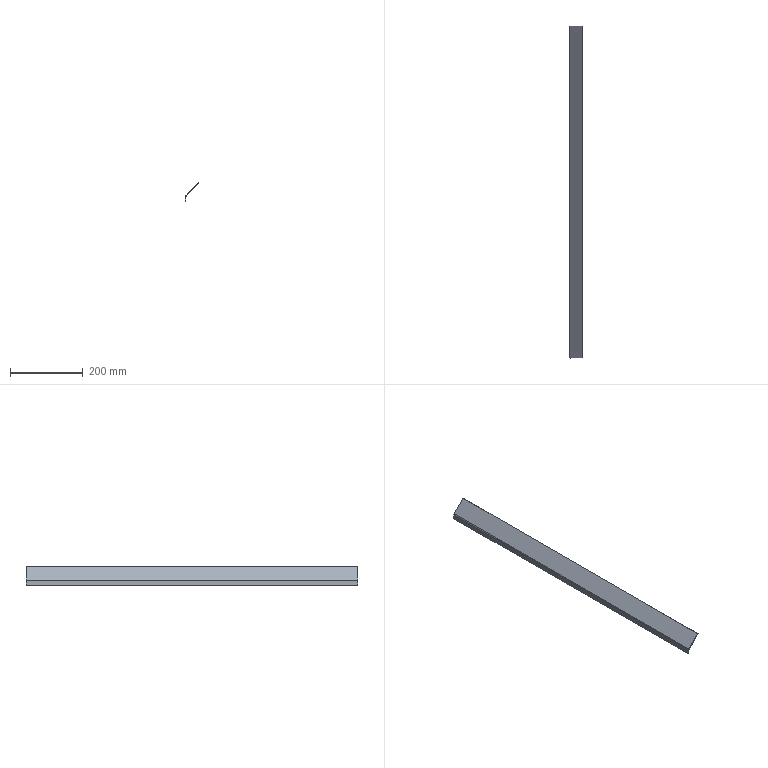Component | SolidWorks | ExhaustVentAssembly-1_Louver-1 | 1 solid | 16 faces | box 37.41 x 914 x 51 mm | volume 118659 mm3 | plane 14 | cylinder 2 | commonest cylinder face diameters 8 x1 4 x1 | material Plain Carbon Steel
STEP:
#1=CARTESIAN_POINT('',(-16.406,6.211,35.255));
#2=VERTEX_POINT('',#1);
#3=CARTESIAN_POINT('',(-16.406,42.1,35.255));
#4=VERTEX_POINT('',#3);
#5=CARTESIAN_POINT('',(-16.406,6.163,35.255));
#6=DIRECTION('',(0.,1.,-0.));
#7=VECTOR('',#6,39.37);
#8=LINE('',#5,#7);
#9=EDGE_CURVE('',#2,#4,#8,.T.);
#10=ORIENTED_EDGE('',*,*,#9,.F.);
#11=CARTESIAN_POINT('',(-16.485,6.211,35.255));
#12=VERTEX_POINT('',#11);
#13=CARTESIAN_POINT('',(-16.406,6.211,35.255));
#14=DIRECTION('',(-1.,0.,-0.));
#15=VECTOR('',#14,39.37);
#16=LINE('',#13,#15);
#17=EDGE_CURVE('',#2,#12,#16,.T.);
#18=ORIENTED_EDGE('',*,*,#17,.T.);
#19=CARTESIAN_POINT('',(-16.485,42.1,35.255));
#20=VERTEX_POINT('',#19);
#21=CARTESIAN_POINT('',(-16.485,6.163,35.255));
#22=DIRECTION('',(0.,1.,-0.));
#23=VECTOR('',#22,39.37);
#24=LINE('',#21,#23);
#25=EDGE_CURVE('',#12,#20,#24,.T.);
#26=ORIENTED_EDGE('',*,*,#25,.T.);
#27=CARTESIAN_POINT('',(-16.406,42.1,35.255));
#28=DIRECTION('',(1.,-0.,0.));
#29=VECTOR('',#28,39.37);
#30=LINE('',#27,#29);
#31=EDGE_CURVE('',#20,#4,#30,.T.);
#32=ORIENTED_EDGE('',*,*,#31,.T.);
#33=EDGE_LOOP('',(#10,#18,#26,#32));
#34=FACE_OUTER_BOUND('',#33,.T.);
#35=CARTESIAN_POINT('',(-16.406,6.163,35.255));
#36=DIRECTION('',(0.,-0.,-1.));
#37=DIRECTION('',(1.,-0.,0.));
#38=AXIS2_PLACEMENT_3D('',#35,#36,#37);
#39=PLANE('',#38);
#40=ADVANCED_FACE('',(#34),#39,.T.);
#41=CARTESIAN_POINT('',(-16.398,6.163,35.815));
#42=VERTEX_POINT('',#41);
#43=CARTESIAN_POINT('',(-16.398,6.163,35.851));
#44=VERTEX_POINT('',#43);
#45=CARTESIAN_POINT('',(-16.398,6.163,35.892));
#46=DIRECTION('',(-0.,0.,1.));
#47=VECTOR('',#46,39.37);
#48=LINE('',#45,#47);
#49=EDGE_CURVE('',#42,#44,#48,.T.);
#50=ORIENTED_EDGE('',*,*,#49,.F.);
#51=CARTESIAN_POINT('',(-16.383,6.163,35.836));
#52=VERTEX_POINT('',#51);
#53=CARTESIAN_POINT('',(-16.327,6.163,35.78));
#54=DIRECTION('',(0.,1.,-0.));
#55=DIRECTION('',(1.,0.,0.));
#56=AXIS2_PLACEMENT_3D('',#53,#54,#55);
#57=CIRCLE('',#56,0.07874);
#58=EDGE_CURVE('',#42,#52,#57,.T.);
#59=ORIENTED_EDGE('',*,*,#58,.T.);
#60=CARTESIAN_POINT('',(-16.439,6.163,35.892));
#61=DIRECTION('',(0.7071,-0.,-0.7071));
#62=VECTOR('',#61,39.37);
#63=LINE('',#60,#62);
#64=EDGE_CURVE('',#44,#52,#63,.T.);
#65=ORIENTED_EDGE('',*,*,#64,.F.);
#66=EDGE_LOOP('',(#50,#59,#65));
#67=FACE_OUTER_BOUND('',#66,.T.);
#68=CARTESIAN_POINT('',(-16.439,6.163,35.892));
#69=DIRECTION('',(-0.,-1.,0.));
#70=DIRECTION('',(1.,-0.,0.));
#71=AXIS2_PLACEMENT_3D('',#68,#69,#70);
#72=PLANE('',#71);
#73=ADVANCED_FACE('',(#67),#72,.T.);
#74=CARTESIAN_POINT('',(-16.398,6.163,35.932));
#75=VERTEX_POINT('',#74);
#76=CARTESIAN_POINT('',(-16.398,6.163,35.78));
#77=DIRECTION('',(-0.,0.,1.));
#78=VECTOR('',#77,39.37);
#79=LINE('',#76,#78);
#80=EDGE_CURVE('',#44,#75,#79,.T.);
#81=ORIENTED_EDGE('',*,*,#80,.F.);
#82=ORIENTED_EDGE('',*,*,#64,.T.);
#83=CARTESIAN_POINT('',(-15.012,6.163,37.207));
#84=VERTEX_POINT('',#83);
#85=CARTESIAN_POINT('',(-16.429,6.163,35.79));
#86=DIRECTION('',(0.7071,0.,0.7071));
#87=VECTOR('',#86,39.37);
#88=LINE('',#85,#87);
#89=EDGE_CURVE('',#52,#84,#88,.T.);
#90=ORIENTED_EDGE('',*,*,#89,.T.);
#91=CARTESIAN_POINT('',(-15.067,6.163,37.263));
#92=VERTEX_POINT('',#91);
#93=CARTESIAN_POINT('',(-15.067,6.163,37.263));
#94=DIRECTION('',(0.7071,-0.,-0.7071));
#95=VECTOR('',#94,39.37);
#96=LINE('',#93,#95);
#97=EDGE_CURVE('',#92,#84,#96,.T.);
#98=ORIENTED_EDGE('',*,*,#97,.F.);
#99=CARTESIAN_POINT('',(-16.485,6.163,35.846));
#100=DIRECTION('',(0.7071,0.,0.7071));
#101=VECTOR('',#100,39.37);
#102=LINE('',#99,#101);
#103=EDGE_CURVE('',#75,#92,#102,.T.);
#104=ORIENTED_EDGE('',*,*,#103,.F.);
#105=EDGE_LOOP('',(#81,#82,#90,#98,#104));
#106=FACE_OUTER_BOUND('',#105,.T.);
#107=CARTESIAN_POINT('',(-16.406,6.163,35.78));
#108=DIRECTION('',(-0.,-1.,0.));
#109=DIRECTION('',(1.,-0.,0.));
#110=AXIS2_PLACEMENT_3D('',#107,#108,#109);
#111=PLANE('',#110);
#112=ADVANCED_FACE('',(#106),#111,.T.);
#113=CARTESIAN_POINT('',(-16.398,42.148,35.851));
#114=VERTEX_POINT('',#113);
#115=CARTESIAN_POINT('',(-16.398,42.148,35.815));
#116=VERTEX_POINT('',#115);
#117=CARTESIAN_POINT('',(-16.398,42.148,35.78));
#118=DIRECTION('',(0.,-0.,-1.));
#119=VECTOR('',#118,39.37);
#120=LINE('',#117,#119);
#121=EDGE_CURVE('',#114,#116,#120,.T.);
#122=ORIENTED_EDGE('',*,*,#121,.F.);
#123=CARTESIAN_POINT('',(-16.383,42.148,35.836));
#124=VERTEX_POINT('',#123);
#125=CARTESIAN_POINT('',(-16.383,42.148,35.836));
#126=DIRECTION('',(-0.7071,0.,0.7071));
#127=VECTOR('',#126,39.37);
#128=LINE('',#125,#127);
#129=EDGE_CURVE('',#124,#114,#128,.T.);
#130=ORIENTED_EDGE('',*,*,#129,.F.);
#131=CARTESIAN_POINT('',(-16.327,42.148,35.78));
#132=DIRECTION('',(0.,1.,-0.));
#133=DIRECTION('',(1.,0.,0.));
#134=AXIS2_PLACEMENT_3D('',#131,#132,#133);
#135=CIRCLE('',#134,0.07874);
#136=EDGE_CURVE('',#116,#124,#135,.T.);
#137=ORIENTED_EDGE('',*,*,#136,.F.);
#138=EDGE_LOOP('',(#122,#130,#137));
#139=FACE_OUTER_BOUND('',#138,.T.);
#140=CARTESIAN_POINT('',(-16.485,42.148,35.78));
#141=DIRECTION('',(0.,1.,-0.));
#142=DIRECTION('',(-1.,0.,-0.));
#143=AXIS2_PLACEMENT_3D('',#140,#141,#142);
#144=PLANE('',#143);
#145=ADVANCED_FACE('',(#139),#144,.T.);
#146=CARTESIAN_POINT('',(-15.012,42.148,37.207));
#147=VERTEX_POINT('',#146);
#148=CARTESIAN_POINT('',(-16.429,42.148,35.79));
#149=DIRECTION('',(0.7071,0.,0.7071));
#150=VECTOR('',#149,39.37);
#151=LINE('',#148,#150);
#152=EDGE_CURVE('',#124,#147,#151,.T.);
#153=ORIENTED_EDGE('',*,*,#152,.T.);
#154=CARTESIAN_POINT('',(-15.012,6.163,37.207));
#155=DIRECTION('',(0.,1.,-0.));
#156=VECTOR('',#155,39.37);
#157=LINE('',#154,#156);
#158=EDGE_CURVE('',#84,#147,#157,.T.);
#159=ORIENTED_EDGE('',*,*,#158,.F.);
#160=ORIENTED_EDGE('',*,*,#89,.F.);
#161=CARTESIAN_POINT('',(-16.383,6.163,35.836));
#162=DIRECTION('',(0.,1.,-0.));
#163=VECTOR('',#162,39.37);
#164=LINE('',#161,#163);
#165=EDGE_CURVE('',#52,#124,#164,.T.);
#166=ORIENTED_EDGE('',*,*,#165,.T.);
#167=EDGE_LOOP('',(#153,#159,#160,#166));
#168=FACE_OUTER_BOUND('',#167,.T.);
#169=CARTESIAN_POINT('',(-16.429,6.163,35.79));
#170=DIRECTION('',(-0.7071,0.,0.7071));
#171=DIRECTION('',(-0.7071,-0.,-0.7071));
#172=AXIS2_PLACEMENT_3D('',#169,#170,#171);
#173=PLANE('',#172);
#174=ADVANCED_FACE('',(#168),#173,.F.);
#175=CARTESIAN_POINT('',(-15.067,42.148,37.263));
#176=VERTEX_POINT('',#175);
#177=CARTESIAN_POINT('',(-15.067,42.148,37.263));
#178=DIRECTION('',(0.7071,-0.,-0.7071));
#179=VECTOR('',#178,39.37);
#180=LINE('',#177,#179);
#181=EDGE_CURVE('',#176,#147,#180,.T.);
#182=ORIENTED_EDGE('',*,*,#181,.F.);
#183=CARTESIAN_POINT('',(-15.067,6.163,37.263));
#184=DIRECTION('',(0.,1.,-0.));
#185=VECTOR('',#184,39.37);
#186=LINE('',#183,#185);
#187=EDGE_CURVE('',#92,#176,#186,.T.);
#188=ORIENTED_EDGE('',*,*,#187,.F.);
#189=ORIENTED_EDGE('',*,*,#97,.T.);
#190=ORIENTED_EDGE('',*,*,#158,.T.);
#191=EDGE_LOOP('',(#182,#188,#189,#190));
#192=FACE_OUTER_BOUND('',#191,.T.);
#193=CARTESIAN_POINT('',(-15.067,6.163,37.263));
#194=DIRECTION('',(0.7071,0.,0.7071));
#195=DIRECTION('',(-0.7071,0.,0.7071));
#196=AXIS2_PLACEMENT_3D('',#193,#194,#195);
#197=PLANE('',#196);
#198=ADVANCED_FACE('',(#192),#197,.T.);
#199=CARTESIAN_POINT('',(-16.398,6.211,35.932));
#200=VERTEX_POINT('',#199);
#201=CARTESIAN_POINT('',(-16.439,6.211,35.892));
#202=VERTEX_POINT('',#201);
#203=CARTESIAN_POINT('',(-16.485,6.211,35.846));
#204=DIRECTION('',(-0.7071,-0.,-0.7071));
#205=VECTOR('',#204,39.37);
#206=LINE('',#203,#205);
#207=EDGE_CURVE('',#200,#202,#206,.T.);
#208=ORIENTED_EDGE('',*,*,#207,.F.);
#209=CARTESIAN_POINT('',(-16.398,6.163,35.932));
#210=DIRECTION('',(0.,1.,-0.));
#211=VECTOR('',#210,39.37);
#212=LINE('',#209,#211);
#213=EDGE_CURVE('',#75,#200,#212,.T.);
#214=ORIENTED_EDGE('',*,*,#213,.F.);
#215=ORIENTED_EDGE('',*,*,#103,.T.);
#216=ORIENTED_EDGE('',*,*,#187,.T.);
#217=CARTESIAN_POINT('',(-16.398,42.148,35.932));
#218=VERTEX_POINT('',#217);
#219=CARTESIAN_POINT('',(-16.485,42.148,35.846));
#220=DIRECTION('',(0.7071,0.,0.7071));
#221=VECTOR('',#220,39.37);
#222=LINE('',#219,#221);
#223=EDGE_CURVE('',#218,#176,#222,.T.);
#224=ORIENTED_EDGE('',*,*,#223,.F.);
#225=CARTESIAN_POINT('',(-16.398,42.1,35.932));
#226=VERTEX_POINT('',#225);
#227=CARTESIAN_POINT('',(-16.398,6.163,35.932));
#228=DIRECTION('',(0.,1.,-0.));
#229=VECTOR('',#228,39.37);
#230=LINE('',#227,#229);
#231=EDGE_CURVE('',#226,#218,#230,.T.);
#232=ORIENTED_EDGE('',*,*,#231,.F.);
#233=CARTESIAN_POINT('',(-16.439,42.1,35.892));
#234=VERTEX_POINT('',#233);
#235=CARTESIAN_POINT('',(-16.485,42.1,35.846));
#236=DIRECTION('',(0.7071,0.,0.7071));
#237=VECTOR('',#236,39.37);
#238=LINE('',#235,#237);
#239=EDGE_CURVE('',#234,#226,#238,.T.);
#240=ORIENTED_EDGE('',*,*,#239,.F.);
#241=CARTESIAN_POINT('',(-16.439,6.163,35.892));
#242=DIRECTION('',(0.,1.,-0.));
#243=VECTOR('',#242,39.37);
#244=LINE('',#241,#243);
#245=EDGE_CURVE('',#202,#234,#244,.T.);
#246=ORIENTED_EDGE('',*,*,#245,.F.);
#247=EDGE_LOOP('',(#208,#214,#215,#216,#224,#232,#240,#246));
#248=FACE_OUTER_BOUND('',#247,.T.);
#249=CARTESIAN_POINT('',(-16.485,6.163,35.846));
#250=DIRECTION('',(-0.7071,0.,0.7071));
#251=DIRECTION('',(-0.7071,-0.,-0.7071));
#252=AXIS2_PLACEMENT_3D('',#249,#250,#251);
#253=PLANE('',#252);
#254=ADVANCED_FACE('',(#248),#253,.T.);
#255=CARTESIAN_POINT('',(-16.485,6.211,35.78));
#256=VERTEX_POINT('',#255);
#257=CARTESIAN_POINT('',(-16.327,6.211,35.78));
#258=DIRECTION('',(-0.,-1.,0.));
#259=DIRECTION('',(-1.,0.,0.));
#260=AXIS2_PLACEMENT_3D('',#257,#258,#259);
#261=CIRCLE('',#260,0.1575);
#262=EDGE_CURVE('',#202,#256,#261,.T.);
#263=ORIENTED_EDGE('',*,*,#262,.F.);
#264=ORIENTED_EDGE('',*,*,#245,.T.);
#265=CARTESIAN_POINT('',(-16.485,42.1,35.78));
#266=VERTEX_POINT('',#265);
#267=CARTESIAN_POINT('',(-16.327,42.1,35.78));
#268=DIRECTION('',(0.,1.,-0.));
#269=DIRECTION('',(1.,0.,0.));
#270=AXIS2_PLACEMENT_3D('',#267,#268,#269);
#271=CIRCLE('',#270,0.1575);
#272=EDGE_CURVE('',#266,#234,#271,.T.);
#273=ORIENTED_EDGE('',*,*,#272,.F.);
#274=CARTESIAN_POINT('',(-16.485,6.163,35.78));
#275=DIRECTION('',(0.,1.,-0.));
#276=VECTOR('',#275,39.37);
#277=LINE('',#274,#276);
#278=EDGE_CURVE('',#256,#266,#277,.T.);
#279=ORIENTED_EDGE('',*,*,#278,.F.);
#280=EDGE_LOOP('',(#263,#264,#273,#279));
#281=FACE_OUTER_BOUND('',#280,.T.);
#282=CARTESIAN_POINT('',(-16.327,6.163,35.78));
#283=DIRECTION('',(0.,1.,-0.));
#284=DIRECTION('',(-1.,0.,0.));
#285=AXIS2_PLACEMENT_3D('',#282,#283,#284);
#286=CYLINDRICAL_SURFACE('',#285,0.1575);
#287=ADVANCED_FACE('',(#281),#286,.T.);
#288=CARTESIAN_POINT('',(-16.485,6.211,35.255));
#289=DIRECTION('',(0.,-0.,-1.));
#290=VECTOR('',#289,39.37);
#291=LINE('',#288,#290);
#292=EDGE_CURVE('',#256,#12,#291,.T.);
#293=ORIENTED_EDGE('',*,*,#292,.F.);
#294=ORIENTED_EDGE('',*,*,#278,.T.);
#295=CARTESIAN_POINT('',(-16.485,42.1,35.255));
#296=DIRECTION('',(-0.,0.,1.));
#297=VECTOR('',#296,39.37);
#298=LINE('',#295,#297);
#299=EDGE_CURVE('',#20,#266,#298,.T.);
#300=ORIENTED_EDGE('',*,*,#299,.F.);
#301=ORIENTED_EDGE('',*,*,#25,.F.);
#302=EDGE_LOOP('',(#293,#294,#300,#301));
#303=FACE_OUTER_BOUND('',#302,.T.);
#304=CARTESIAN_POINT('',(-16.485,6.163,35.255));
#305=DIRECTION('',(-1.,0.,-0.));
#306=DIRECTION('',(-0.,-1.,0.));
#307=AXIS2_PLACEMENT_3D('',#304,#305,#306);
#308=PLANE('',#307);
#309=ADVANCED_FACE('',(#303),#308,.T.);
#310=CARTESIAN_POINT('',(-16.406,6.211,35.78));
#311=VERTEX_POINT('',#310);
#312=CARTESIAN_POINT('',(-16.406,42.1,35.78));
#313=VERTEX_POINT('',#312);
#314=CARTESIAN_POINT('',(-16.406,6.163,35.78));
#315=DIRECTION('',(0.,1.,-0.));
#316=VECTOR('',#315,39.37);
#317=LINE('',#314,#316);
#318=EDGE_CURVE('',#311,#313,#317,.T.);
#319=ORIENTED_EDGE('',*,*,#318,.F.);
#320=CARTESIAN_POINT('',(-16.406,6.211,35.255));
#321=DIRECTION('',(0.,-0.,-1.));
#322=VECTOR('',#321,39.37);
#323=LINE('',#320,#322);
#324=EDGE_CURVE('',#311,#2,#323,.T.);
#325=ORIENTED_EDGE('',*,*,#324,.T.);
#326=ORIENTED_EDGE('',*,*,#9,.T.);
#327=CARTESIAN_POINT('',(-16.406,42.1,35.255));
#328=DIRECTION('',(-0.,0.,1.));
#329=VECTOR('',#328,39.37);
#330=LINE('',#327,#329);
#331=EDGE_CURVE('',#4,#313,#330,.T.);
#332=ORIENTED_EDGE('',*,*,#331,.T.);
#333=EDGE_LOOP('',(#319,#325,#326,#332));
#334=FACE_OUTER_BOUND('',#333,.T.);
#335=CARTESIAN_POINT('',(-16.406,6.163,35.255));
#336=DIRECTION('',(-1.,0.,-0.));
#337=DIRECTION('',(-0.,-1.,0.));
#338=AXIS2_PLACEMENT_3D('',#335,#336,#337);
#339=PLANE('',#338);
#340=ADVANCED_FACE('',(#334),#339,.F.);
#341=CARTESIAN_POINT('',(-16.398,6.211,35.815));
#342=VERTEX_POINT('',#341);
#343=CARTESIAN_POINT('',(-16.398,6.163,35.815));
#344=DIRECTION('',(0.,1.,-0.));
#345=VECTOR('',#344,39.37);
#346=LINE('',#343,#345);
#347=EDGE_CURVE('',#42,#342,#346,.T.);
#348=ORIENTED_EDGE('',*,*,#347,.T.);
#349=CARTESIAN_POINT('',(-16.327,6.211,35.78));
#350=DIRECTION('',(-0.,-1.,0.));
#351=DIRECTION('',(-1.,0.,0.));
#352=AXIS2_PLACEMENT_3D('',#349,#350,#351);
#353=CIRCLE('',#352,0.07874);
#354=EDGE_CURVE('',#342,#311,#353,.T.);
#355=ORIENTED_EDGE('',*,*,#354,.T.);
#356=ORIENTED_EDGE('',*,*,#318,.T.);
#357=CARTESIAN_POINT('',(-16.398,42.1,35.815));
#358=VERTEX_POINT('',#357);
#359=CARTESIAN_POINT('',(-16.327,42.1,35.78));
#360=DIRECTION('',(0.,1.,-0.));
#361=DIRECTION('',(1.,0.,-0.));
#362=AXIS2_PLACEMENT_3D('',#359,#360,#361);
#363=CIRCLE('',#362,0.07874);
#364=EDGE_CURVE('',#313,#358,#363,.T.);
#365=ORIENTED_EDGE('',*,*,#364,.T.);
#366=CARTESIAN_POINT('',(-16.398,6.163,35.815));
#367=DIRECTION('',(0.,1.,-0.));
#368=VECTOR('',#367,39.37);
#369=LINE('',#366,#368);
#370=EDGE_CURVE('',#358,#116,#369,.T.);
#371=ORIENTED_EDGE('',*,*,#370,.T.);
#372=ORIENTED_EDGE('',*,*,#136,.T.);
#373=ORIENTED_EDGE('',*,*,#165,.F.);
#374=ORIENTED_EDGE('',*,*,#58,.F.);
#375=EDGE_LOOP('',(#348,#355,#356,#365,#371,#372,#373,#374));
#376=FACE_OUTER_BOUND('',#375,.T.);
#377=CARTESIAN_POINT('',(-16.327,6.163,35.78));
#378=DIRECTION('',(0.,1.,-0.));
#379=DIRECTION('',(-1.,0.,0.));
#380=AXIS2_PLACEMENT_3D('',#377,#378,#379);
#381=CYLINDRICAL_SURFACE('',#380,0.07874);
#382=ADVANCED_FACE('',(#376),#381,.F.);
#383=ORIENTED_EDGE('',*,*,#129,.T.);
#384=CARTESIAN_POINT('',(-16.398,42.148,35.78));
#385=DIRECTION('',(-0.,0.,1.));
#386=VECTOR('',#385,39.37);
#387=LINE('',#384,#386);
#388=EDGE_CURVE('',#114,#218,#387,.T.);
#389=ORIENTED_EDGE('',*,*,#388,.T.);
#390=ORIENTED_EDGE('',*,*,#223,.T.);
#391=ORIENTED_EDGE('',*,*,#181,.T.);
#392=ORIENTED_EDGE('',*,*,#152,.F.);
#393=EDGE_LOOP('',(#383,#389,#390,#391,#392));
#394=FACE_OUTER_BOUND('',#393,.T.);
#395=CARTESIAN_POINT('',(-16.327,42.148,35.78));
#396=DIRECTION('',(-0.,-1.,0.));
#397=DIRECTION('',(1.,-0.,0.));
#398=AXIS2_PLACEMENT_3D('',#395,#396,#397);
#399=PLANE('',#398);
#400=ADVANCED_FACE('',(#394),#399,.F.);
#401=ORIENTED_EDGE('',*,*,#239,.T.);
#402=CARTESIAN_POINT('',(-16.398,42.1,35.255));
#403=DIRECTION('',(-0.,0.,1.));
#404=VECTOR('',#403,39.37);
#405=LINE('',#402,#404);
#406=EDGE_CURVE('',#358,#226,#405,.T.);
#407=ORIENTED_EDGE('',*,*,#406,.F.);
#408=ORIENTED_EDGE('',*,*,#364,.F.);
#409=ORIENTED_EDGE('',*,*,#331,.F.);
#410=ORIENTED_EDGE('',*,*,#31,.F.);
#411=ORIENTED_EDGE('',*,*,#299,.T.);
#412=ORIENTED_EDGE('',*,*,#272,.T.);
#413=EDGE_LOOP('',(#401,#407,#408,#409,#410,#411,#412));
#414=FACE_OUTER_BOUND('',#413,.T.);
#415=CARTESIAN_POINT('',(-16.398,42.1,35.255));
#416=DIRECTION('',(-0.,-1.,0.));
#417=DIRECTION('',(1.,-0.,0.));
#418=AXIS2_PLACEMENT_3D('',#415,#416,#417);
#419=PLANE('',#418);
#420=ADVANCED_FACE('',(#414),#419,.F.);
#421=ORIENTED_EDGE('',*,*,#406,.T.);
#422=ORIENTED_EDGE('',*,*,#231,.T.);
#423=ORIENTED_EDGE('',*,*,#388,.F.);
#424=ORIENTED_EDGE('',*,*,#121,.T.);
#425=ORIENTED_EDGE('',*,*,#370,.F.);
#426=EDGE_LOOP('',(#421,#422,#423,#424,#425));
#427=FACE_OUTER_BOUND('',#426,.T.);
#428=CARTESIAN_POINT('',(-16.398,42.177,35.255));
#429=DIRECTION('',(1.,-0.,0.));
#430=DIRECTION('',(0.,1.,-0.));
#431=AXIS2_PLACEMENT_3D('',#428,#429,#430);
#432=PLANE('',#431);
#433=ADVANCED_FACE('',(#427),#432,.F.);
#434=ORIENTED_EDGE('',*,*,#207,.T.);
#435=ORIENTED_EDGE('',*,*,#262,.T.);
#436=ORIENTED_EDGE('',*,*,#292,.T.);
#437=ORIENTED_EDGE('',*,*,#17,.F.);
#438=ORIENTED_EDGE('',*,*,#324,.F.);
#439=ORIENTED_EDGE('',*,*,#354,.F.);
#440=CARTESIAN_POINT('',(-16.398,6.211,35.255));
#441=DIRECTION('',(-0.,0.,1.));
#442=VECTOR('',#441,39.37);
#443=LINE('',#440,#442);
#444=EDGE_CURVE('',#342,#200,#443,.T.);
#445=ORIENTED_EDGE('',*,*,#444,.T.);
#446=EDGE_LOOP('',(#434,#435,#436,#437,#438,#439,#445));
#447=FACE_OUTER_BOUND('',#446,.T.);
#448=CARTESIAN_POINT('',(-16.398,6.211,35.255));
#449=DIRECTION('',(0.,1.,-0.));
#450=DIRECTION('',(-1.,0.,-0.));
#451=AXIS2_PLACEMENT_3D('',#448,#449,#450);
#452=PLANE('',#451);
#453=ADVANCED_FACE('',(#447),#452,.F.);
#454=ORIENTED_EDGE('',*,*,#213,.T.);
#455=ORIENTED_EDGE('',*,*,#444,.F.);
#456=ORIENTED_EDGE('',*,*,#347,.F.);
#457=ORIENTED_EDGE('',*,*,#49,.T.);
#458=ORIENTED_EDGE('',*,*,#80,.T.);
#459=EDGE_LOOP('',(#454,#455,#456,#457,#458));
#460=FACE_OUTER_BOUND('',#459,.T.);
#461=CARTESIAN_POINT('',(-16.398,6.211,35.255));
#462=DIRECTION('',(1.,-0.,0.));
#463=DIRECTION('',(0.,1.,-0.));
#464=AXIS2_PLACEMENT_3D('',#461,#462,#463);
#465=PLANE('',#464);
#466=ADVANCED_FACE('',(#460),#465,.F.);
#467=CLOSED_SHELL('',(#40,#73,#112,#145,#174,#198,#254,#287,#309,#340,#382,#400,#420,#433,#453,#466));
#468=MANIFOLD_SOLID_BREP('',#467);
#469=CARTESIAN_POINT('',(0.,0.,0.));
#470=DIRECTION('',(0.,0.,1.));
#471=DIRECTION('',(1.,0.,0.));
#472=AXIS2_PLACEMENT_3D('',#469,#470,#471);
#473=(LENGTH_UNIT()NAMED_UNIT(*)SI_UNIT($,.METRE.));
#474=LENGTH_MEASURE_WITH_UNIT(LENGTH_MEASURE(0.0254),#473);
#475=DIMENSIONAL_EXPONENTS(1.,0.,0.,0.,0.,0.,0.);
#476=(CONVERSION_BASED_UNIT('',#474)LENGTH_UNIT()NAMED_UNIT(#475));
#477=UNCERTAINTY_MEASURE_WITH_UNIT(LENGTH_MEASURE(0.00001),#476,'','');
#478=(NAMED_UNIT(*)PLANE_ANGLE_UNIT()SI_UNIT($,.RADIAN.));
#479=(NAMED_UNIT(*)SI_UNIT($,.STERADIAN.)SOLID_ANGLE_UNIT());
#480=(GEOMETRIC_REPRESENTATION_CONTEXT(3)GLOBAL_UNCERTAINTY_ASSIGNED_CONTEXT((#477))GLOBAL_UNIT_ASSIGNED_CONTEXT((#476,#478,#479))REPRESENTATION_CONTEXT('',''));
#481=ADVANCED_BREP_SHAPE_REPRESENTATION('',(#468,#472),#480);
#482=COLOUR_RGB('',0.7922,0.8196,0.9333);
#483=FILL_AREA_STYLE_COLOUR('',#482);
#484=FILL_AREA_STYLE('',(#483));
#485=SURFACE_STYLE_FILL_AREA(#484);
#486=SURFACE_SIDE_STYLE('',(#485));
#487=SURFACE_STYLE_USAGE(.BOTH.,#486);
#488=PRESENTATION_STYLE_ASSIGNMENT((#487));
#489=STYLED_ITEM('',(#488),#468);
#490=(LENGTH_UNIT()NAMED_UNIT(*)SI_UNIT($,.METRE.));
#491=LENGTH_MEASURE_WITH_UNIT(LENGTH_MEASURE(0.0254),#490);
#492=DIMENSIONAL_EXPONENTS(1.,0.,0.,0.,0.,0.,0.);
#493=(CONVERSION_BASED_UNIT('',#491)LENGTH_UNIT()NAMED_UNIT(#492));
#494=UNCERTAINTY_MEASURE_WITH_UNIT(LENGTH_MEASURE(0.00001),#493,'','');
#495=(NAMED_UNIT(*)PLANE_ANGLE_UNIT()SI_UNIT($,.RADIAN.));
#496=(NAMED_UNIT(*)SI_UNIT($,.STERADIAN.)SOLID_ANGLE_UNIT());
#497=(GEOMETRIC_REPRESENTATION_CONTEXT(3)GLOBAL_UNCERTAINTY_ASSIGNED_CONTEXT((#494))GLOBAL_UNIT_ASSIGNED_CONTEXT((#493,#495,#496))REPRESENTATION_CONTEXT('',''));
#498=MECHANICAL_DESIGN_GEOMETRIC_PRESENTATION_REPRESENTATION('',(#489),#497);
#499=PRESENTATION_LAYER_ASSIGNMENT('','',(#489));